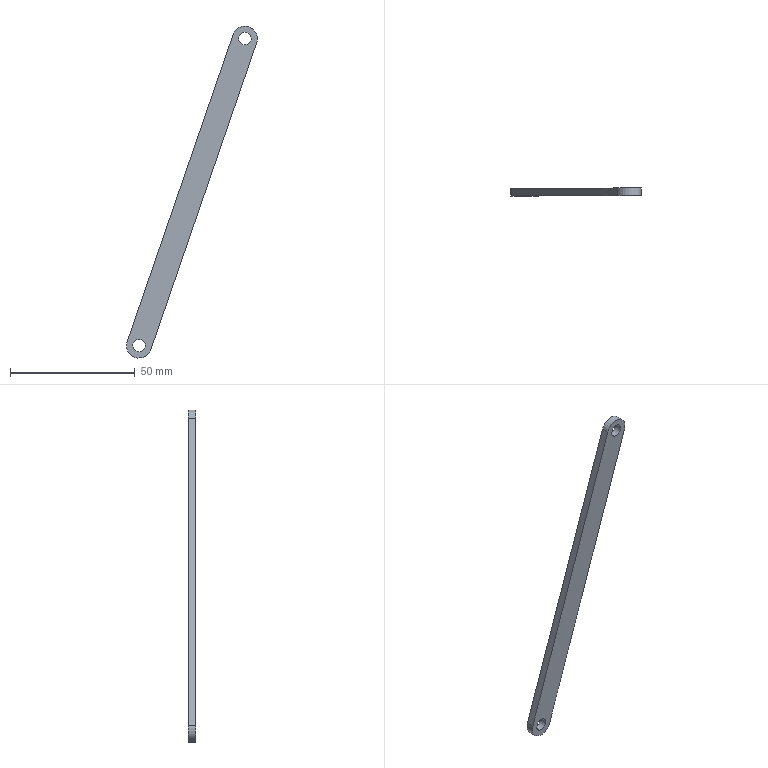Component | SolidWorks | WheelAssembly2-1_ConnectingRod3-1 | 1 solid | 11 faces | box 52.37 x 3 x 132.9 mm | volume 4018 mm3 | cylinder 7 | plane 4 | commonest cylinder face diameters 5 x4 10 x3
build123d program:
from build123d import *

# Parameters (mm, degrees)
SKETCH1_R           = 2.5
BOSS_EXTRUDE1_DEPTH = 3


with BuildPart() as part:
    # Sketch1 → Boss-Extrude1 (new body)
    with BuildSketch(Plane.XY):
        with BuildLine():
            Line((-65, 5), (65, 5))
            ThreePointArc((65, 5), (70, 0), (65, -5))
            Line((65, -5), (-65, -5))
            ThreePointArc((-65, -5), (-70, 0), (-65, 5))
        make_face()
        with Locations((-65, 0)):
            Circle(SKETCH1_R, mode=Mode.SUBTRACT)
        with Locations((65, 0)):
            Circle(SKETCH1_R, mode=Mode.SUBTRACT)
    extrude(amount=BOSS_EXTRUDE1_DEPTH)


solid = part.part

# Placed as in the assembly
solid = solid.moved(Location((-249.773, -33, -391.519), (-90, 0, -70.98)))
STEP:
#1=COLOUR_RGB('',0.7922,0.8196,0.9333);
#2=FILL_AREA_STYLE_COLOUR('',#1);
#3=FILL_AREA_STYLE('',(#2));
#4=SURFACE_STYLE_FILL_AREA(#3);
#5=SURFACE_SIDE_STYLE('',(#4));
#6=SURFACE_STYLE_USAGE(.BOTH.,#5);
#7=PRESENTATION_STYLE_ASSIGNMENT((#6));
#8=CARTESIAN_POINT('',(-9.032,-1.299,-13.088));
#9=VERTEX_POINT('',#8);
#10=CARTESIAN_POINT('',(-8.968,-1.299,-12.902));
#11=VERTEX_POINT('',#10);
#12=CARTESIAN_POINT('',(-9.,-1.299,-12.995));
#13=DIRECTION('',(0.,-1.,-0.));
#14=DIRECTION('',(0.3259,0.,0.9454));
#15=AXIS2_PLACEMENT_3D('',#12,#13,#14);
#16=CIRCLE('',#15,0.09843);
#17=EDGE_CURVE('',#9,#11,#16,.T.);
#18=ORIENTED_EDGE('',*,*,#17,.T.);
#19=CARTESIAN_POINT('',(-8.968,-1.181,-12.902));
#20=VERTEX_POINT('',#19);
#21=CARTESIAN_POINT('',(-8.968,-1.299,-12.902));
#22=DIRECTION('',(-0.,1.,0.));
#23=VECTOR('',#22,39.37);
#24=LINE('',#21,#23);
#25=EDGE_CURVE('',#11,#20,#24,.T.);
#26=ORIENTED_EDGE('',*,*,#25,.T.);
#27=CARTESIAN_POINT('',(-9.032,-1.181,-13.088));
#28=VERTEX_POINT('',#27);
#29=CARTESIAN_POINT('',(-9.,-1.181,-12.995));
#30=DIRECTION('',(0.,-1.,-0.));
#31=DIRECTION('',(0.3259,0.,0.9454));
#32=AXIS2_PLACEMENT_3D('',#29,#30,#31);
#33=CIRCLE('',#32,0.09843);
#34=EDGE_CURVE('',#28,#20,#33,.T.);
#35=ORIENTED_EDGE('',*,*,#34,.F.);
#36=CARTESIAN_POINT('',(-9.032,-1.299,-13.088));
#37=DIRECTION('',(-0.,1.,0.));
#38=VECTOR('',#37,39.37);
#39=LINE('',#36,#38);
#40=EDGE_CURVE('',#9,#28,#39,.T.);
#41=ORIENTED_EDGE('',*,*,#40,.F.);
#42=EDGE_LOOP('',(#18,#26,#35,#41));
#43=FACE_OUTER_BOUND('',#42,.T.);
#44=CARTESIAN_POINT('',(-9.,-1.299,-12.995));
#45=DIRECTION('',(-0.,1.,0.));
#46=DIRECTION('',(-0.3259,0.,-0.9454));
#47=AXIS2_PLACEMENT_3D('',#44,#45,#46);
#48=CYLINDRICAL_SURFACE('',#47,0.09843);
#49=ADVANCED_FACE('',(#43),#48,.F.);
#50=CARTESIAN_POINT('',(-10.7,-1.299,-17.927));
#51=VERTEX_POINT('',#50);
#52=CARTESIAN_POINT('',(-10.635,-1.299,-17.74));
#53=VERTEX_POINT('',#52);
#54=CARTESIAN_POINT('',(-10.668,-1.299,-17.833));
#55=DIRECTION('',(0.,-1.,-0.));
#56=DIRECTION('',(0.3259,0.,0.9454));
#57=AXIS2_PLACEMENT_3D('',#54,#55,#56);
#58=CIRCLE('',#57,0.09843);
#59=EDGE_CURVE('',#51,#53,#58,.T.);
#60=ORIENTED_EDGE('',*,*,#59,.T.);
#61=CARTESIAN_POINT('',(-10.635,-1.181,-17.74));
#62=VERTEX_POINT('',#61);
#63=CARTESIAN_POINT('',(-10.635,-1.299,-17.74));
#64=DIRECTION('',(-0.,1.,0.));
#65=VECTOR('',#64,39.37);
#66=LINE('',#63,#65);
#67=EDGE_CURVE('',#53,#62,#66,.T.);
#68=ORIENTED_EDGE('',*,*,#67,.T.);
#69=CARTESIAN_POINT('',(-10.7,-1.181,-17.927));
#70=VERTEX_POINT('',#69);
#71=CARTESIAN_POINT('',(-10.668,-1.181,-17.833));
#72=DIRECTION('',(0.,-1.,-0.));
#73=DIRECTION('',(0.3259,0.,0.9454));
#74=AXIS2_PLACEMENT_3D('',#71,#72,#73);
#75=CIRCLE('',#74,0.09843);
#76=EDGE_CURVE('',#70,#62,#75,.T.);
#77=ORIENTED_EDGE('',*,*,#76,.F.);
#78=CARTESIAN_POINT('',(-10.7,-1.299,-17.927));
#79=DIRECTION('',(-0.,1.,0.));
#80=VECTOR('',#79,39.37);
#81=LINE('',#78,#80);
#82=EDGE_CURVE('',#51,#70,#81,.T.);
#83=ORIENTED_EDGE('',*,*,#82,.F.);
#84=EDGE_LOOP('',(#60,#68,#77,#83));
#85=FACE_OUTER_BOUND('',#84,.T.);
#86=CARTESIAN_POINT('',(-10.668,-1.299,-17.833));
#87=DIRECTION('',(-0.,1.,0.));
#88=DIRECTION('',(-0.3259,0.,-0.9454));
#89=AXIS2_PLACEMENT_3D('',#86,#87,#88);
#90=CYLINDRICAL_SURFACE('',#89,0.09843);
#91=ADVANCED_FACE('',(#85),#90,.F.);
#92=CARTESIAN_POINT('',(-10.732,-1.299,-18.02));
#93=VERTEX_POINT('',#92);
#94=CARTESIAN_POINT('',(-10.481,-1.299,-17.898));
#95=VERTEX_POINT('',#94);
#96=CARTESIAN_POINT('',(-10.668,-1.299,-17.833));
#97=DIRECTION('',(0.,-1.,-0.));
#98=DIRECTION('',(0.3259,0.,0.9454));
#99=AXIS2_PLACEMENT_3D('',#96,#97,#98);
#100=CIRCLE('',#99,0.1969);
#101=EDGE_CURVE('',#93,#95,#100,.T.);
#102=ORIENTED_EDGE('',*,*,#101,.F.);
#103=CARTESIAN_POINT('',(-10.732,-1.181,-18.02));
#104=VERTEX_POINT('',#103);
#105=CARTESIAN_POINT('',(-10.732,-1.299,-18.02));
#106=DIRECTION('',(-0.,1.,0.));
#107=VECTOR('',#106,39.37);
#108=LINE('',#105,#107);
#109=EDGE_CURVE('',#93,#104,#108,.T.);
#110=ORIENTED_EDGE('',*,*,#109,.T.);
#111=CARTESIAN_POINT('',(-10.481,-1.181,-17.898));
#112=VERTEX_POINT('',#111);
#113=CARTESIAN_POINT('',(-10.668,-1.181,-17.833));
#114=DIRECTION('',(0.,-1.,-0.));
#115=DIRECTION('',(0.3259,0.,0.9454));
#116=AXIS2_PLACEMENT_3D('',#113,#114,#115);
#117=CIRCLE('',#116,0.1969);
#118=EDGE_CURVE('',#104,#112,#117,.T.);
#119=ORIENTED_EDGE('',*,*,#118,.T.);
#120=CARTESIAN_POINT('',(-10.481,-1.299,-17.898));
#121=DIRECTION('',(-0.,1.,0.));
#122=VECTOR('',#121,39.37);
#123=LINE('',#120,#122);
#124=EDGE_CURVE('',#95,#112,#123,.T.);
#125=ORIENTED_EDGE('',*,*,#124,.F.);
#126=EDGE_LOOP('',(#102,#110,#119,#125));
#127=FACE_OUTER_BOUND('',#126,.T.);
#128=CARTESIAN_POINT('',(-10.668,-1.299,-17.833));
#129=DIRECTION('',(-0.,1.,0.));
#130=DIRECTION('',(-0.3259,0.,-0.9454));
#131=AXIS2_PLACEMENT_3D('',#128,#129,#130);
#132=CYLINDRICAL_SURFACE('',#131,0.1969);
#133=ADVANCED_FACE('',(#127),#132,.T.);
#134=ORIENTED_EDGE('',*,*,#59,.F.);
#135=CARTESIAN_POINT('',(-10.668,-1.299,-17.833));
#136=DIRECTION('',(0.,-1.,-0.));
#137=DIRECTION('',(0.3259,0.,0.9454));
#138=AXIS2_PLACEMENT_3D('',#135,#136,#137);
#139=CIRCLE('',#138,0.09843);
#140=EDGE_CURVE('',#53,#51,#139,.T.);
#141=ORIENTED_EDGE('',*,*,#140,.F.);
#142=EDGE_LOOP('',(#134,#141));
#143=FACE_BOUND('',#142,.T.);
#144=CARTESIAN_POINT('',(-10.854,-1.299,-17.769));
#145=VERTEX_POINT('',#144);
#146=CARTESIAN_POINT('',(-10.668,-1.299,-17.833));
#147=DIRECTION('',(0.,-1.,-0.));
#148=DIRECTION('',(0.3259,0.,0.9454));
#149=AXIS2_PLACEMENT_3D('',#146,#147,#148);
#150=CIRCLE('',#149,0.1969);
#151=EDGE_CURVE('',#145,#93,#150,.T.);
#152=ORIENTED_EDGE('',*,*,#151,.T.);
#153=ORIENTED_EDGE('',*,*,#101,.T.);
#154=CARTESIAN_POINT('',(-8.813,-1.299,-13.059));
#155=VERTEX_POINT('',#154);
#156=CARTESIAN_POINT('',(-10.481,-1.299,-17.898));
#157=DIRECTION('',(0.3259,0.,0.9454));
#158=VECTOR('',#157,39.37);
#159=LINE('',#156,#158);
#160=EDGE_CURVE('',#95,#155,#159,.T.);
#161=ORIENTED_EDGE('',*,*,#160,.T.);
#162=CARTESIAN_POINT('',(-9.186,-1.299,-12.931));
#163=VERTEX_POINT('',#162);
#164=CARTESIAN_POINT('',(-9.,-1.299,-12.995));
#165=DIRECTION('',(0.,-1.,-0.));
#166=DIRECTION('',(0.3259,0.,0.9454));
#167=AXIS2_PLACEMENT_3D('',#164,#165,#166);
#168=CIRCLE('',#167,0.1969);
#169=EDGE_CURVE('',#155,#163,#168,.T.);
#170=ORIENTED_EDGE('',*,*,#169,.T.);
#171=CARTESIAN_POINT('',(-10.854,-1.299,-17.769));
#172=DIRECTION('',(-0.3259,-0.,-0.9454));
#173=VECTOR('',#172,39.37);
#174=LINE('',#171,#173);
#175=EDGE_CURVE('',#163,#145,#174,.T.);
#176=ORIENTED_EDGE('',*,*,#175,.T.);
#177=EDGE_LOOP('',(#152,#153,#161,#170,#176));
#178=FACE_OUTER_BOUND('',#177,.T.);
#179=ORIENTED_EDGE('',*,*,#17,.F.);
#180=CARTESIAN_POINT('',(-9.,-1.299,-12.995));
#181=DIRECTION('',(0.,-1.,-0.));
#182=DIRECTION('',(0.3259,0.,0.9454));
#183=AXIS2_PLACEMENT_3D('',#180,#181,#182);
#184=CIRCLE('',#183,0.09843);
#185=EDGE_CURVE('',#11,#9,#184,.T.);
#186=ORIENTED_EDGE('',*,*,#185,.F.);
#187=EDGE_LOOP('',(#179,#186));
#188=FACE_BOUND('',#187,.T.);
#189=CARTESIAN_POINT('',(-10.668,-1.299,-17.833));
#190=DIRECTION('',(0.,-1.,-0.));
#191=DIRECTION('',(0.3259,0.,0.9454));
#192=AXIS2_PLACEMENT_3D('',#189,#190,#191);
#193=PLANE('',#192);
#194=ADVANCED_FACE('',(#143,#178,#188),#193,.T.);
#195=CARTESIAN_POINT('',(-10.854,-1.181,-17.769));
#196=VERTEX_POINT('',#195);
#197=CARTESIAN_POINT('',(-10.668,-1.181,-17.833));
#198=DIRECTION('',(0.,-1.,-0.));
#199=DIRECTION('',(0.3259,0.,0.9454));
#200=AXIS2_PLACEMENT_3D('',#197,#198,#199);
#201=CIRCLE('',#200,0.1969);
#202=EDGE_CURVE('',#196,#104,#201,.T.);
#203=ORIENTED_EDGE('',*,*,#202,.F.);
#204=CARTESIAN_POINT('',(-9.186,-1.181,-12.931));
#205=VERTEX_POINT('',#204);
#206=CARTESIAN_POINT('',(-10.854,-1.181,-17.769));
#207=DIRECTION('',(-0.3259,-0.,-0.9454));
#208=VECTOR('',#207,39.37);
#209=LINE('',#206,#208);
#210=EDGE_CURVE('',#205,#196,#209,.T.);
#211=ORIENTED_EDGE('',*,*,#210,.F.);
#212=CARTESIAN_POINT('',(-8.813,-1.181,-13.059));
#213=VERTEX_POINT('',#212);
#214=CARTESIAN_POINT('',(-9.,-1.181,-12.995));
#215=DIRECTION('',(0.,-1.,-0.));
#216=DIRECTION('',(0.3259,0.,0.9454));
#217=AXIS2_PLACEMENT_3D('',#214,#215,#216);
#218=CIRCLE('',#217,0.1969);
#219=EDGE_CURVE('',#213,#205,#218,.T.);
#220=ORIENTED_EDGE('',*,*,#219,.F.);
#221=CARTESIAN_POINT('',(-10.481,-1.181,-17.898));
#222=DIRECTION('',(0.3259,0.,0.9454));
#223=VECTOR('',#222,39.37);
#224=LINE('',#221,#223);
#225=EDGE_CURVE('',#112,#213,#224,.T.);
#226=ORIENTED_EDGE('',*,*,#225,.F.);
#227=ORIENTED_EDGE('',*,*,#118,.F.);
#228=EDGE_LOOP('',(#203,#211,#220,#226,#227));
#229=FACE_OUTER_BOUND('',#228,.T.);
#230=ORIENTED_EDGE('',*,*,#76,.T.);
#231=CARTESIAN_POINT('',(-10.668,-1.181,-17.833));
#232=DIRECTION('',(0.,-1.,-0.));
#233=DIRECTION('',(0.3259,0.,0.9454));
#234=AXIS2_PLACEMENT_3D('',#231,#232,#233);
#235=CIRCLE('',#234,0.09843);
#236=EDGE_CURVE('',#62,#70,#235,.T.);
#237=ORIENTED_EDGE('',*,*,#236,.T.);
#238=EDGE_LOOP('',(#230,#237));
#239=FACE_BOUND('',#238,.T.);
#240=ORIENTED_EDGE('',*,*,#34,.T.);
#241=CARTESIAN_POINT('',(-9.,-1.181,-12.995));
#242=DIRECTION('',(0.,-1.,-0.));
#243=DIRECTION('',(0.3259,0.,0.9454));
#244=AXIS2_PLACEMENT_3D('',#241,#242,#243);
#245=CIRCLE('',#244,0.09843);
#246=EDGE_CURVE('',#20,#28,#245,.T.);
#247=ORIENTED_EDGE('',*,*,#246,.T.);
#248=EDGE_LOOP('',(#240,#247));
#249=FACE_BOUND('',#248,.T.);
#250=CARTESIAN_POINT('',(-10.668,-1.181,-17.833));
#251=DIRECTION('',(0.,-1.,-0.));
#252=DIRECTION('',(0.3259,0.,0.9454));
#253=AXIS2_PLACEMENT_3D('',#250,#251,#252);
#254=PLANE('',#253);
#255=ADVANCED_FACE('',(#229,#239,#249),#254,.F.);
#256=ORIENTED_EDGE('',*,*,#109,.F.);
#257=ORIENTED_EDGE('',*,*,#151,.F.);
#258=CARTESIAN_POINT('',(-10.854,-1.299,-17.769));
#259=DIRECTION('',(-0.,1.,0.));
#260=VECTOR('',#259,39.37);
#261=LINE('',#258,#260);
#262=EDGE_CURVE('',#145,#196,#261,.T.);
#263=ORIENTED_EDGE('',*,*,#262,.T.);
#264=ORIENTED_EDGE('',*,*,#202,.T.);
#265=EDGE_LOOP('',(#256,#257,#263,#264));
#266=FACE_OUTER_BOUND('',#265,.T.);
#267=CARTESIAN_POINT('',(-10.668,-1.299,-17.833));
#268=DIRECTION('',(-0.,1.,0.));
#269=DIRECTION('',(-0.3259,0.,-0.9454));
#270=AXIS2_PLACEMENT_3D('',#267,#268,#269);
#271=CYLINDRICAL_SURFACE('',#270,0.1969);
#272=ADVANCED_FACE('',(#266),#271,.T.);
#273=ORIENTED_EDGE('',*,*,#225,.T.);
#274=CARTESIAN_POINT('',(-8.813,-1.299,-13.059));
#275=DIRECTION('',(-0.,1.,0.));
#276=VECTOR('',#275,39.37);
#277=LINE('',#274,#276);
#278=EDGE_CURVE('',#155,#213,#277,.T.);
#279=ORIENTED_EDGE('',*,*,#278,.F.);
#280=ORIENTED_EDGE('',*,*,#160,.F.);
#281=ORIENTED_EDGE('',*,*,#124,.T.);
#282=EDGE_LOOP('',(#273,#279,#280,#281));
#283=FACE_OUTER_BOUND('',#282,.T.);
#284=CARTESIAN_POINT('',(-10.481,-1.299,-17.898));
#285=DIRECTION('',(-0.9454,-0.,0.3259));
#286=DIRECTION('',(0.,-1.,-0.));
#287=AXIS2_PLACEMENT_3D('',#284,#285,#286);
#288=PLANE('',#287);
#289=ADVANCED_FACE('',(#283),#288,.F.);
#290=ORIENTED_EDGE('',*,*,#219,.T.);
#291=CARTESIAN_POINT('',(-9.186,-1.299,-12.931));
#292=DIRECTION('',(-0.,1.,0.));
#293=VECTOR('',#292,39.37);
#294=LINE('',#291,#293);
#295=EDGE_CURVE('',#163,#205,#294,.T.);
#296=ORIENTED_EDGE('',*,*,#295,.F.);
#297=ORIENTED_EDGE('',*,*,#169,.F.);
#298=ORIENTED_EDGE('',*,*,#278,.T.);
#299=EDGE_LOOP('',(#290,#296,#297,#298));
#300=FACE_OUTER_BOUND('',#299,.T.);
#301=CARTESIAN_POINT('',(-9.,-1.299,-12.995));
#302=DIRECTION('',(-0.,1.,0.));
#303=DIRECTION('',(-0.3259,0.,-0.9454));
#304=AXIS2_PLACEMENT_3D('',#301,#302,#303);
#305=CYLINDRICAL_SURFACE('',#304,0.1969);
#306=ADVANCED_FACE('',(#300),#305,.T.);
#307=ORIENTED_EDGE('',*,*,#210,.T.);
#308=ORIENTED_EDGE('',*,*,#262,.F.);
#309=ORIENTED_EDGE('',*,*,#175,.F.);
#310=ORIENTED_EDGE('',*,*,#295,.T.);
#311=EDGE_LOOP('',(#307,#308,#309,#310));
#312=FACE_OUTER_BOUND('',#311,.T.);
#313=CARTESIAN_POINT('',(-10.854,-1.299,-17.769));
#314=DIRECTION('',(0.9454,0.,-0.3259));
#315=DIRECTION('',(-0.,1.,0.));
#316=AXIS2_PLACEMENT_3D('',#313,#314,#315);
#317=PLANE('',#316);
#318=ADVANCED_FACE('',(#312),#317,.F.);
#319=ORIENTED_EDGE('',*,*,#67,.F.);
#320=ORIENTED_EDGE('',*,*,#140,.T.);
#321=ORIENTED_EDGE('',*,*,#82,.T.);
#322=ORIENTED_EDGE('',*,*,#236,.F.);
#323=EDGE_LOOP('',(#319,#320,#321,#322));
#324=FACE_OUTER_BOUND('',#323,.T.);
#325=CARTESIAN_POINT('',(-10.668,-1.299,-17.833));
#326=DIRECTION('',(-0.,1.,0.));
#327=DIRECTION('',(-0.3259,0.,-0.9454));
#328=AXIS2_PLACEMENT_3D('',#325,#326,#327);
#329=CYLINDRICAL_SURFACE('',#328,0.09843);
#330=ADVANCED_FACE('',(#324),#329,.F.);
#331=ORIENTED_EDGE('',*,*,#25,.F.);
#332=ORIENTED_EDGE('',*,*,#185,.T.);
#333=ORIENTED_EDGE('',*,*,#40,.T.);
#334=ORIENTED_EDGE('',*,*,#246,.F.);
#335=EDGE_LOOP('',(#331,#332,#333,#334));
#336=FACE_OUTER_BOUND('',#335,.T.);
#337=CARTESIAN_POINT('',(-9.,-1.299,-12.995));
#338=DIRECTION('',(-0.,1.,0.));
#339=DIRECTION('',(-0.3259,0.,-0.9454));
#340=AXIS2_PLACEMENT_3D('',#337,#338,#339);
#341=CYLINDRICAL_SURFACE('',#340,0.09843);
#342=ADVANCED_FACE('',(#336),#341,.F.);
#343=CLOSED_SHELL('',(#49,#91,#133,#194,#255,#272,#289,#306,#318,#330,#342));
#344=MANIFOLD_SOLID_BREP('',#343);
#345=STYLED_ITEM('',(#7),#344);
#346=PRESENTATION_LAYER_ASSIGNMENT('','',(#345));
#347=CARTESIAN_POINT('',(0.,0.,0.));
#348=DIRECTION('',(0.,0.,1.));
#349=DIRECTION('',(1.,0.,0.));
#350=AXIS2_PLACEMENT_3D('',#347,#348,#349);
#351=(LENGTH_UNIT()NAMED_UNIT(*)SI_UNIT($,.METRE.));
#352=LENGTH_MEASURE_WITH_UNIT(LENGTH_MEASURE(0.0254),#351);
#353=DIMENSIONAL_EXPONENTS(1.,0.,0.,0.,0.,0.,0.);
#354=(CONVERSION_BASED_UNIT('',#352)LENGTH_UNIT()NAMED_UNIT(#353));
#355=UNCERTAINTY_MEASURE_WITH_UNIT(LENGTH_MEASURE(0.00001),#354,'','');
#356=(NAMED_UNIT(*)PLANE_ANGLE_UNIT()SI_UNIT($,.RADIAN.));
#357=(NAMED_UNIT(*)SI_UNIT($,.STERADIAN.)SOLID_ANGLE_UNIT());
#358=(GEOMETRIC_REPRESENTATION_CONTEXT(3)GLOBAL_UNCERTAINTY_ASSIGNED_CONTEXT((#355))GLOBAL_UNIT_ASSIGNED_CONTEXT((#354,#356,#357))REPRESENTATION_CONTEXT('',''));
#359=ADVANCED_BREP_SHAPE_REPRESENTATION('',(#344,#350),#358);
#360=(LENGTH_UNIT()NAMED_UNIT(*)SI_UNIT($,.METRE.));
#361=LENGTH_MEASURE_WITH_UNIT(LENGTH_MEASURE(0.0254),#360);
#362=DIMENSIONAL_EXPONENTS(1.,0.,0.,0.,0.,0.,0.);
#363=(CONVERSION_BASED_UNIT('',#361)LENGTH_UNIT()NAMED_UNIT(#362));
#364=UNCERTAINTY_MEASURE_WITH_UNIT(LENGTH_MEASURE(0.00001),#363,'','');
#365=(NAMED_UNIT(*)PLANE_ANGLE_UNIT()SI_UNIT($,.RADIAN.));
#366=(NAMED_UNIT(*)SI_UNIT($,.STERADIAN.)SOLID_ANGLE_UNIT());
#367=(GEOMETRIC_REPRESENTATION_CONTEXT(3)GLOBAL_UNCERTAINTY_ASSIGNED_CONTEXT((#364))GLOBAL_UNIT_ASSIGNED_CONTEXT((#363,#365,#366))REPRESENTATION_CONTEXT('',''));
#368=MECHANICAL_DESIGN_GEOMETRIC_PRESENTATION_REPRESENTATION('',(#345),#367);